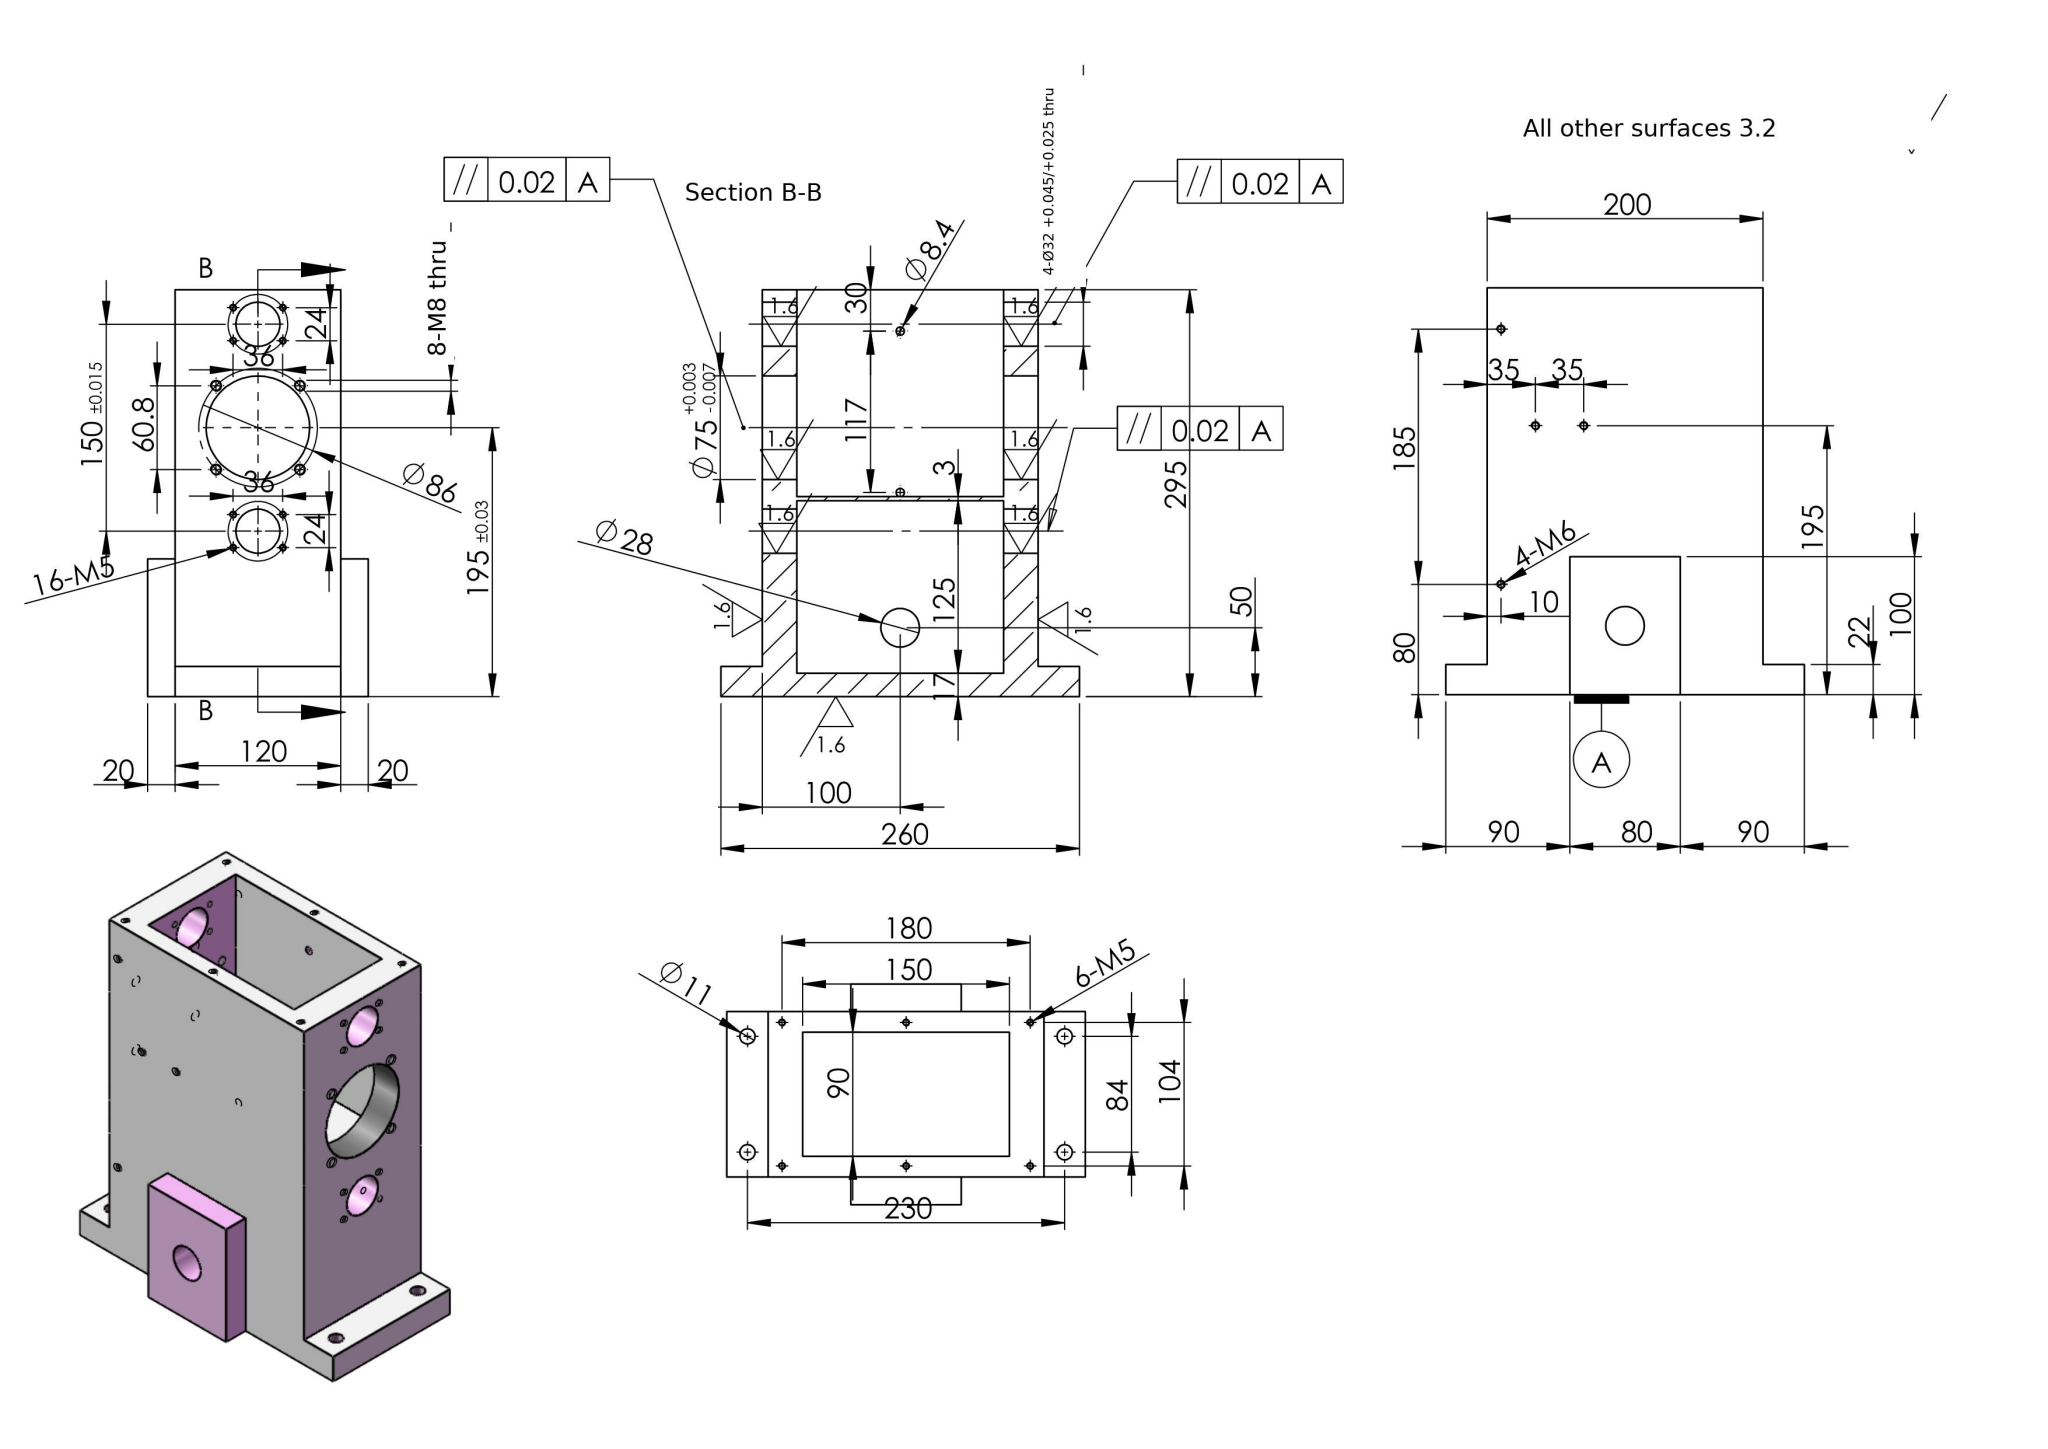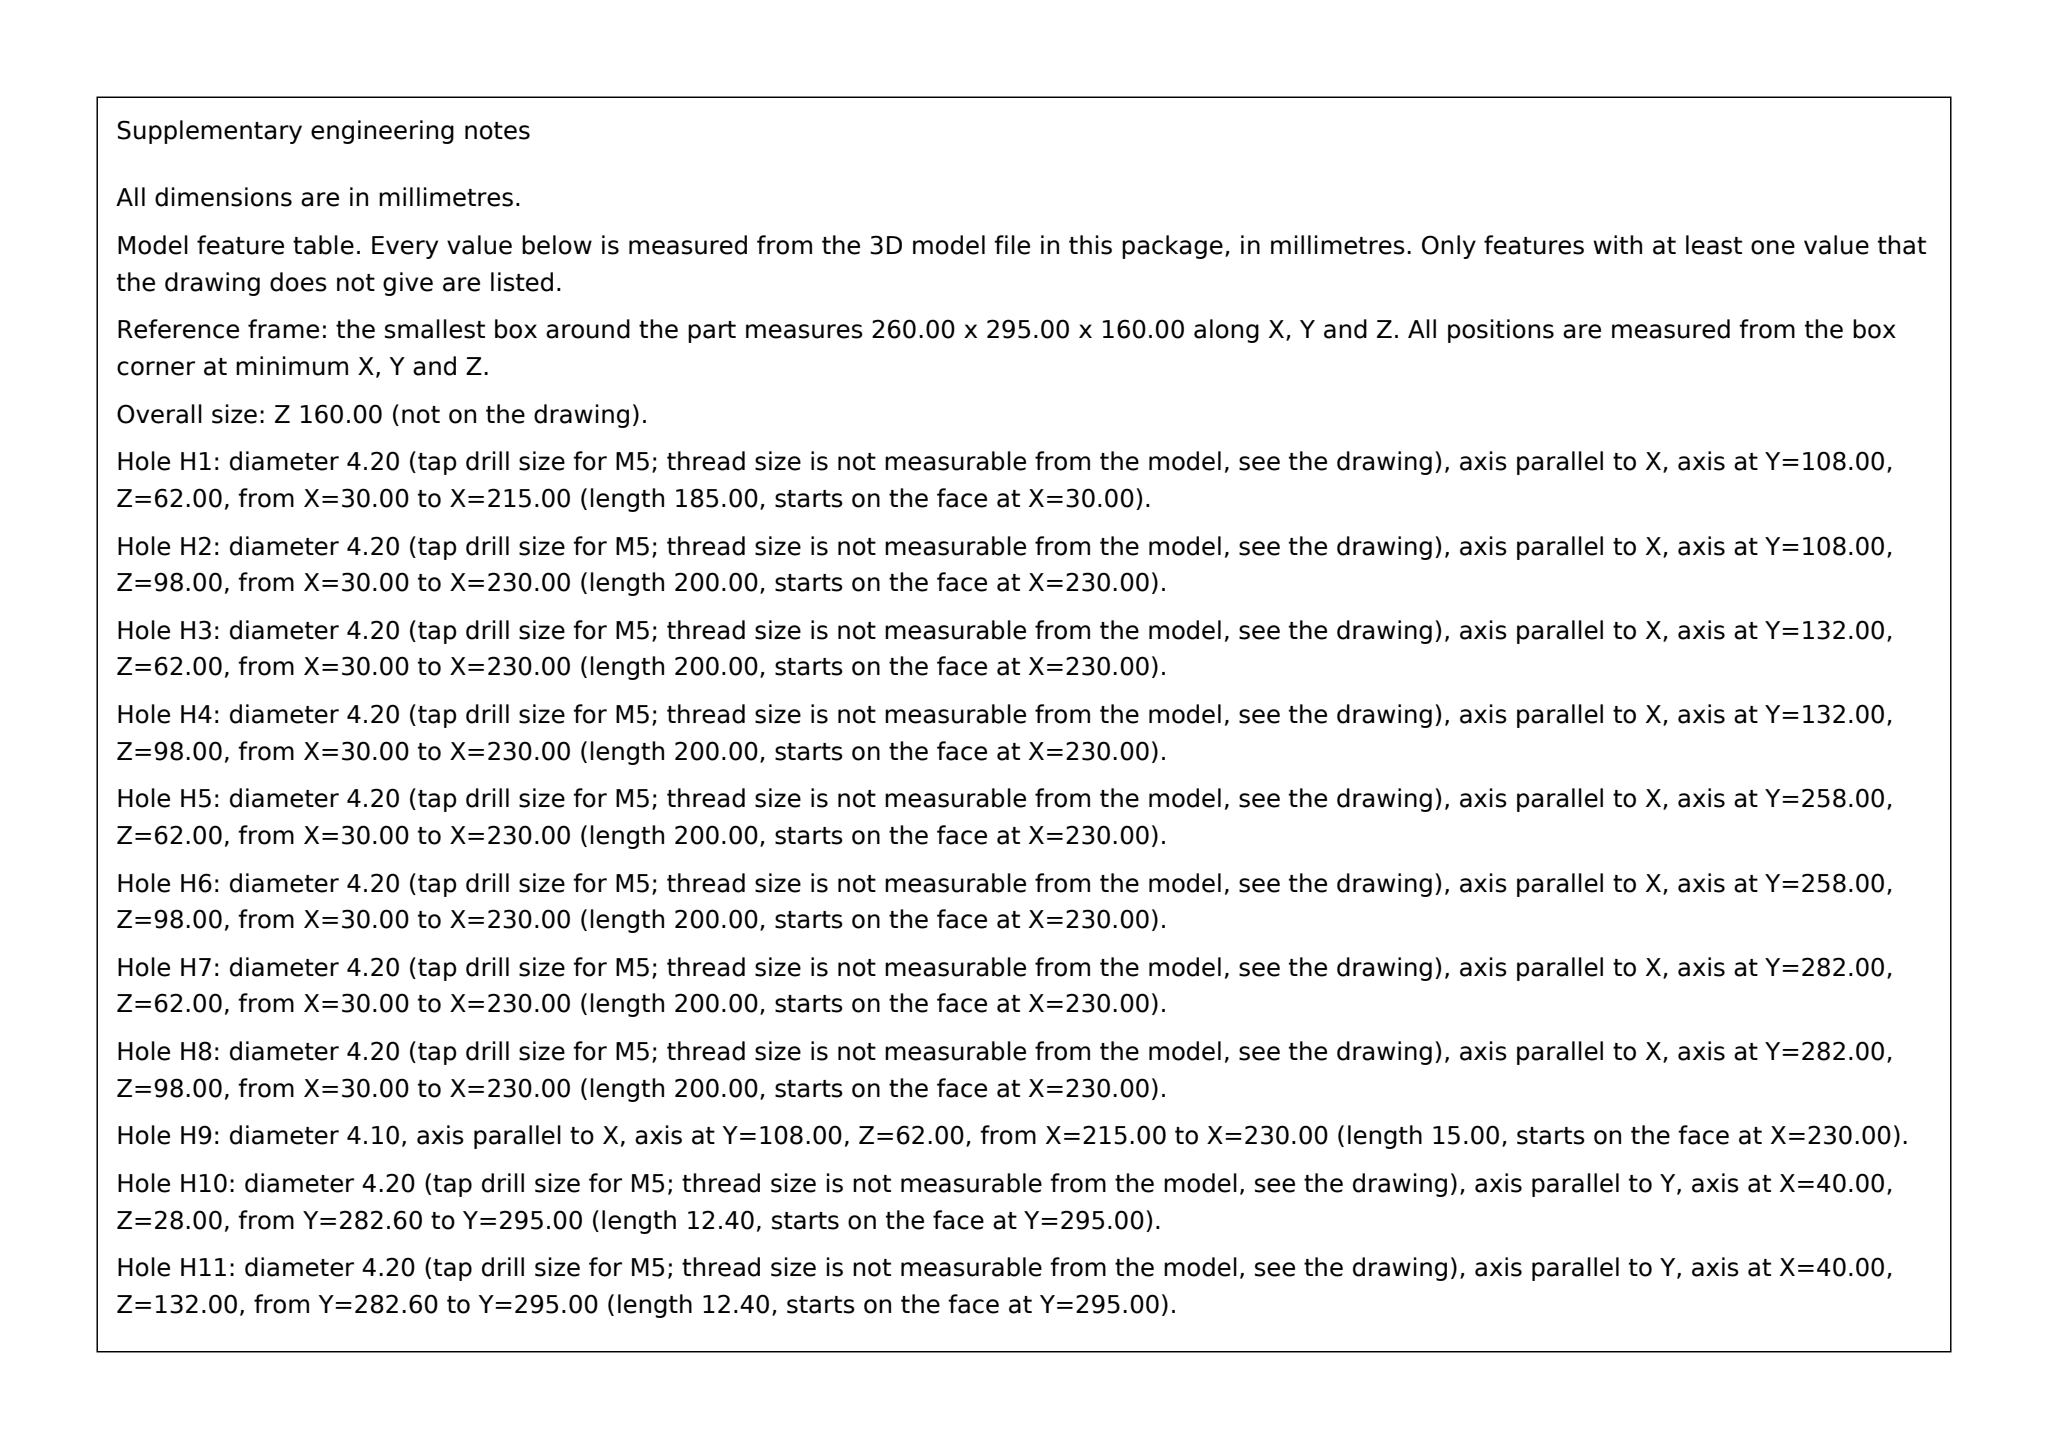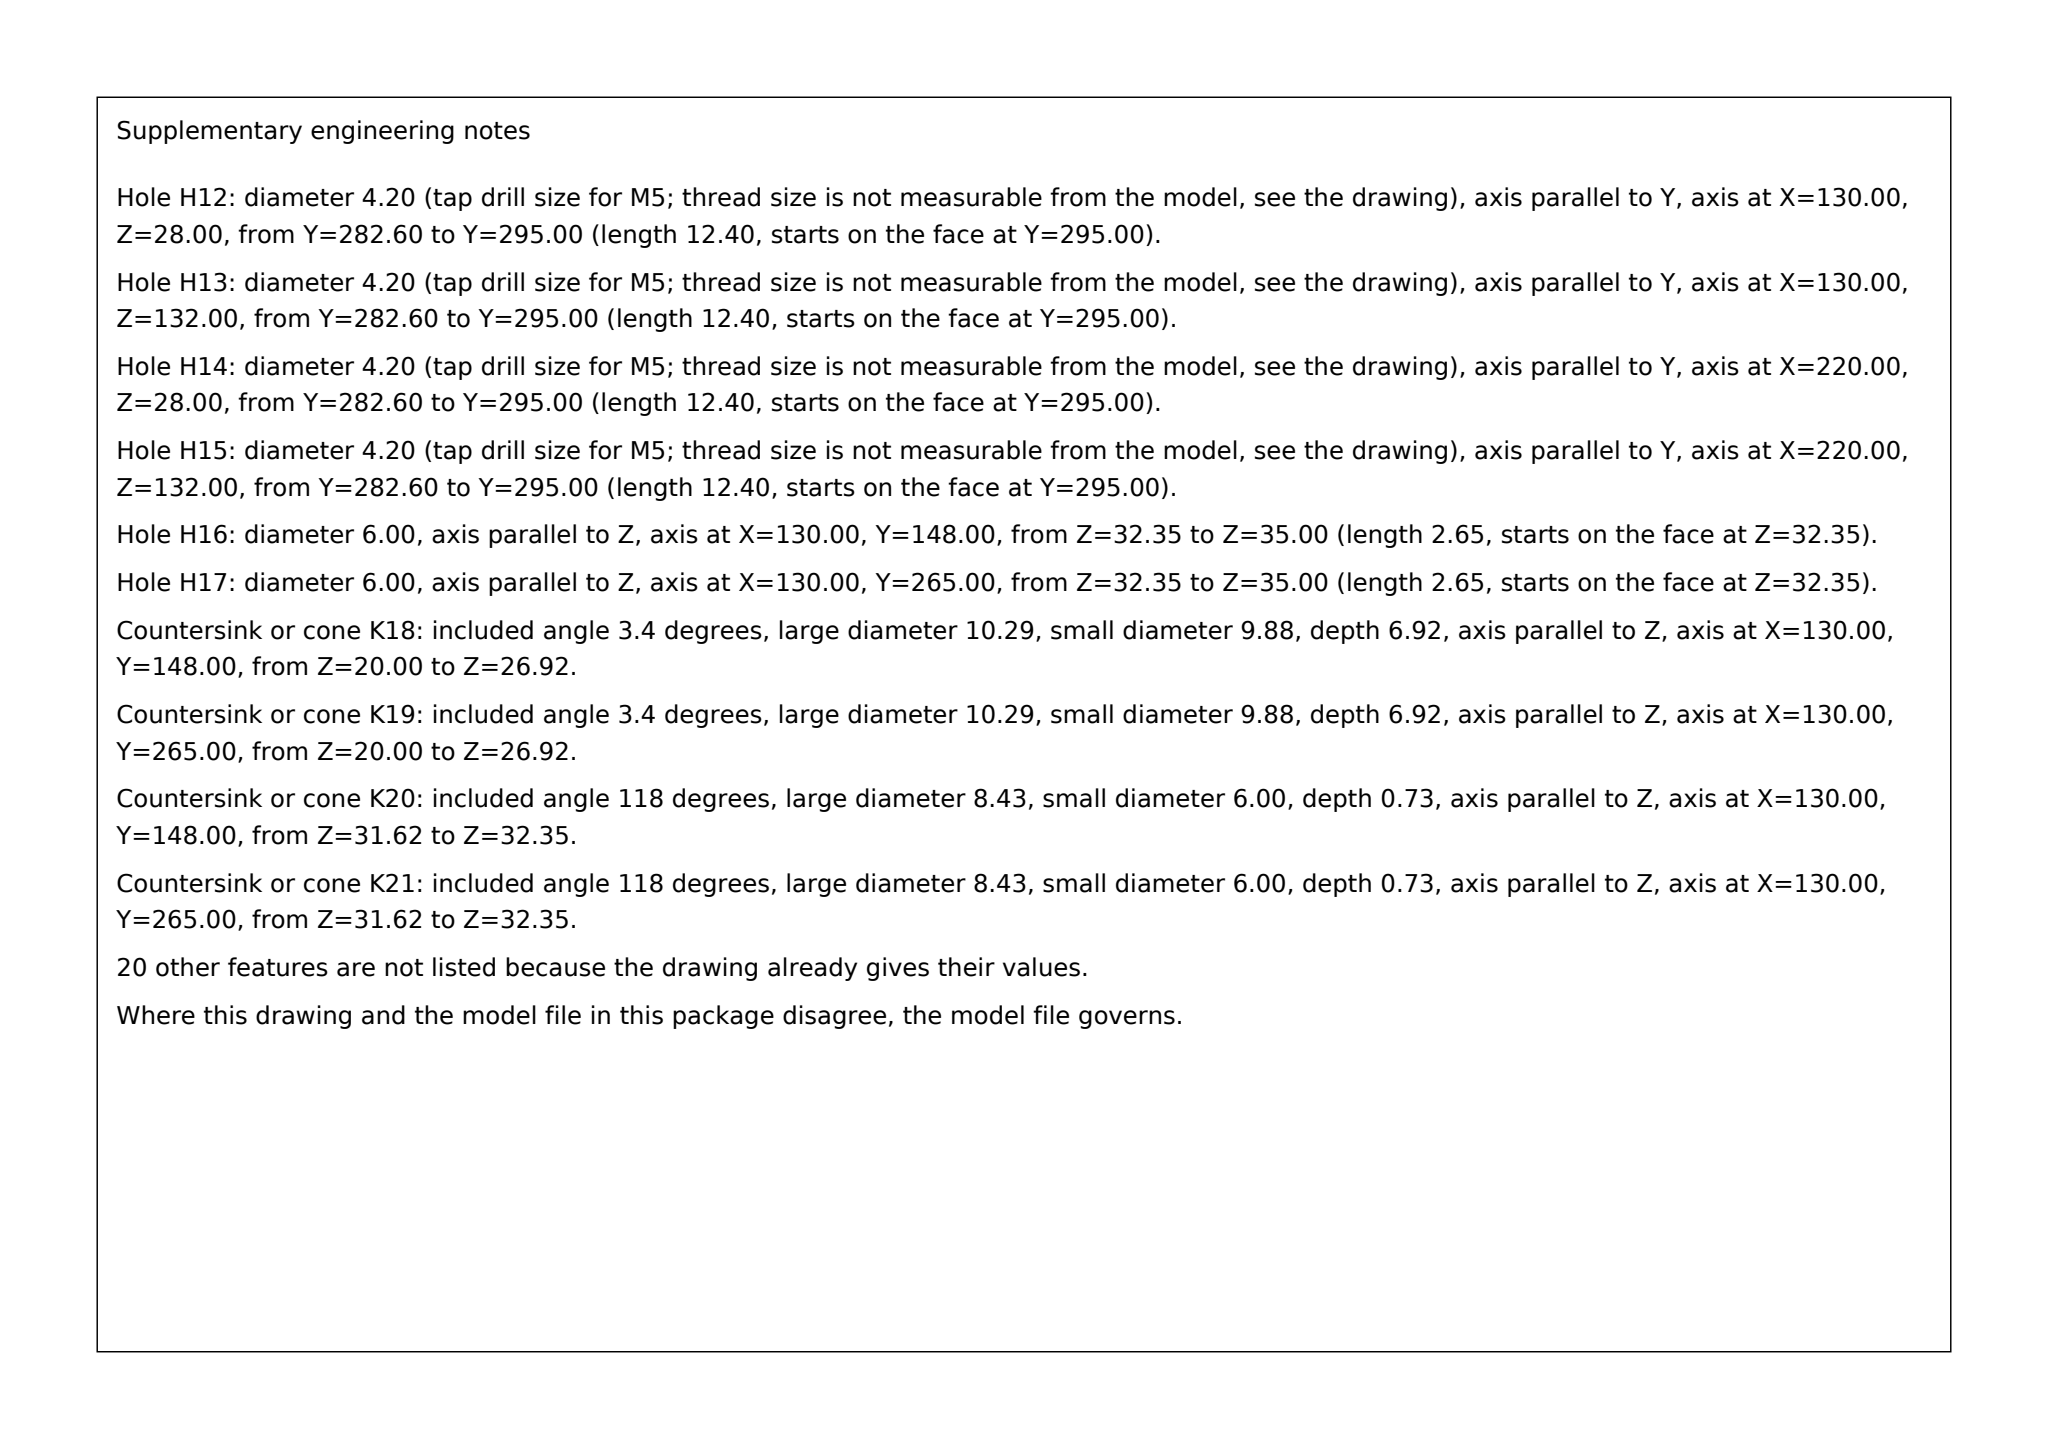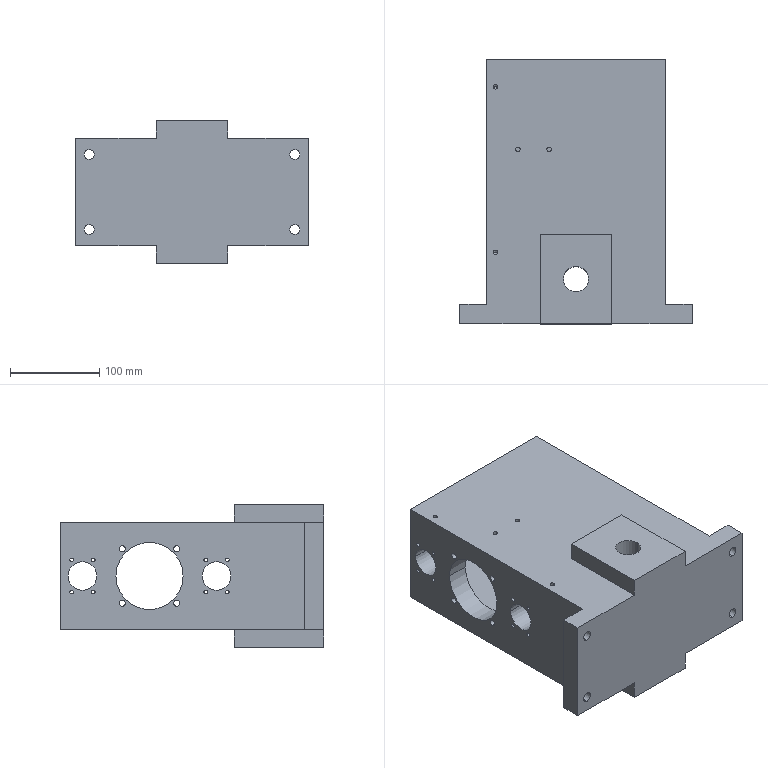Part | SolidWorks | mm | 1 solid | 166 faces | box 260 x 295 x 160 mm | volume 3475609 mm3 | cylinder 106 | plane 32 | cone 28 | commonest cylinder face diameters 4.2 x44 6.8 x16 5 x12 32 x8 11 x8 28 x4 8.433 x4 6 x4